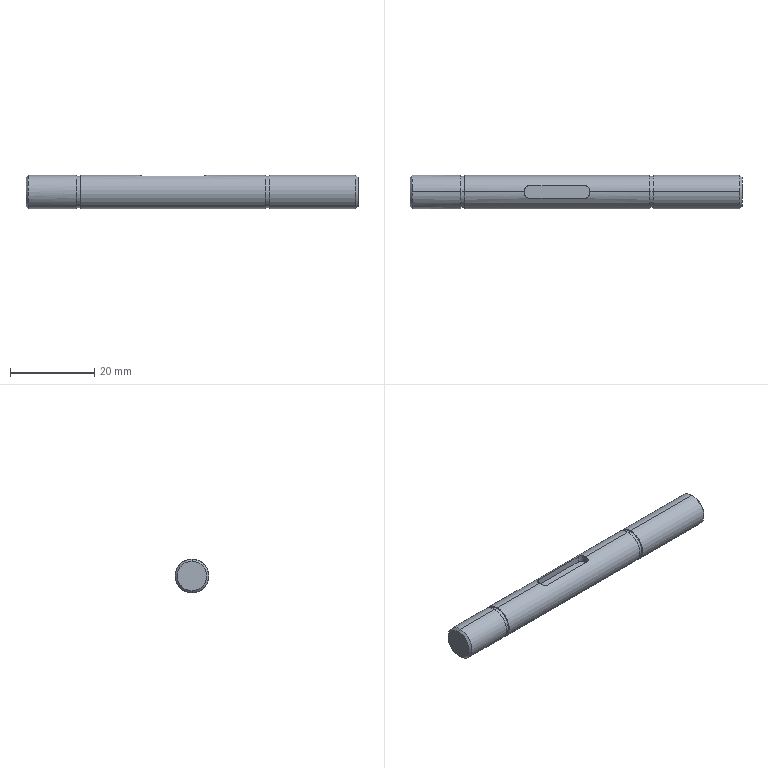CAM job | Mastercam | mm | 3 operations | part box 79 x 8 x 8
1. Contour (Ramp) | 1 - 2 平铣刀
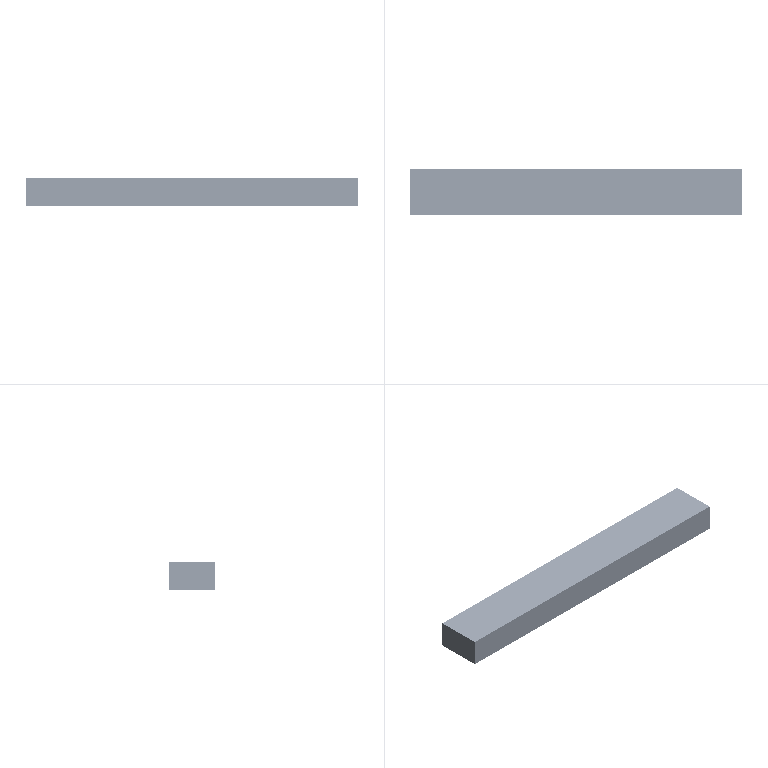2. Contour (2D) | 2 - 2 平铣刀
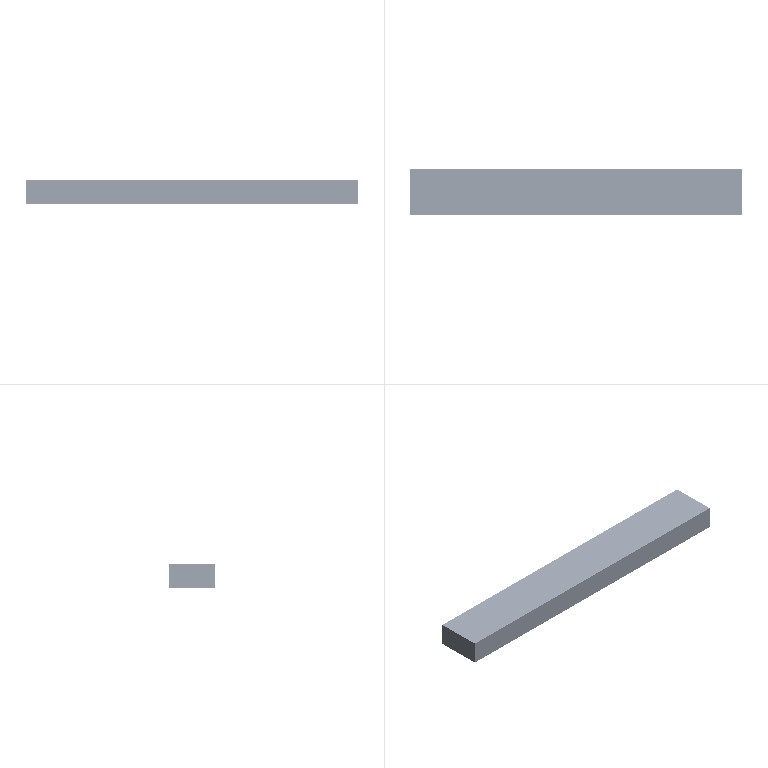3. Contour (3D chamfer) | 3 - 4 倒角刀